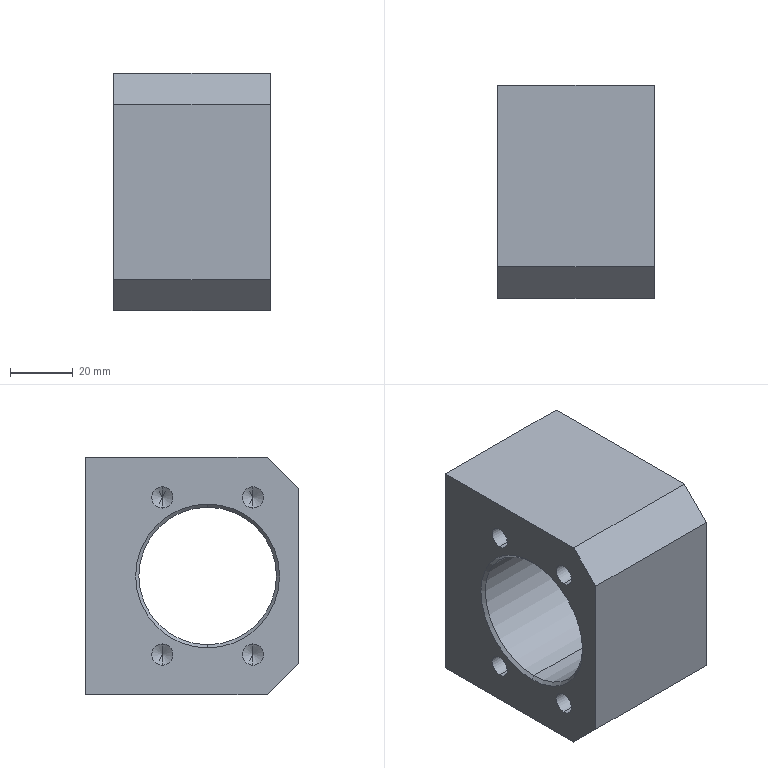Component | SolidWorks | TC020.05-04-1 | 1 solid | 46 faces | volume 172528 mm3 | cone 20 | cylinder 18 | plane 8 | commonest cylinder face diameters 5 x8 6.8 x8 44 x2 | material Q235A